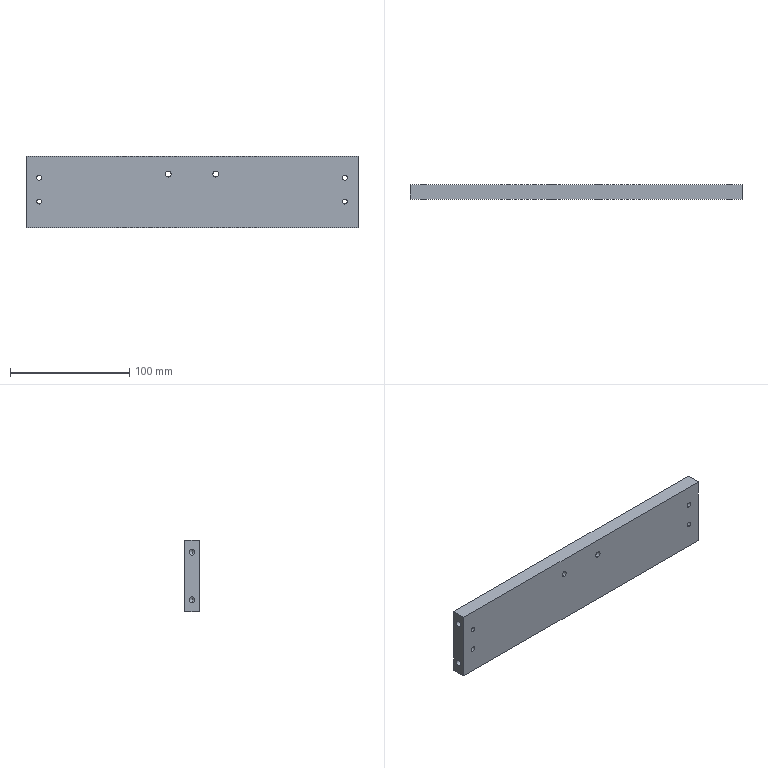Component | SolidWorks | OPW-05-005-1 | 1 solid | 34 faces | box 278 x 12 x 60 mm | volume 197649 mm3 | cylinder 20 | cone 8 | plane 6 | commonest cylinder face diameters 5 x12 4.2 x8
build123d program:
from build123d import *

# Parameters (mm, degrees)
SKETCH1_W                  = 278
SKETCH1_H                  = 60
BOSS_EXTRUDE1_DEPTH        = 6
M6_TAPPED_HOLE1_AT_2_COUNT = 2
M6_TAPPED_HOLE1_AT_2_PITCH = 40
M5_TAPPED_HOLE1_D          = 4.2
M5_TAPPED_HOLE1_DEPTH      = 14
M5_TAPPED_HOLE1_TIP        = 1.262
M6_TAPPED_HOLE2_D          = 5
M6_TAPPED_HOLE2_DEPTH      = 17
M6_TAPPED_HOLE2_TIP        = 1.502


with BuildPart() as part:
    # Sketch1 → Boss-Extrude1 (new, symmetric)
    with BuildSketch(Plane(origin=(0, 0, 0), x_dir=(1, 0, 0), z_dir=(0, 1, 0))):
        Rectangle(SKETCH1_W, SKETCH1_H)
    extrude(amount=BOSS_EXTRUDE1_DEPTH, both=True)

    # Sketch4 → M6 Tapped Hole1 (revolve, cut)
    with BuildSketch(Plane(origin=(-139, 0, -20), x_dir=(0, 0, 1), z_dir=(0, 1, 0))):
        Polygon((0, 0), (0, 18.502), (2.5, 17), (2.5, 0), align=None)
    m6_tapped_hole1 = revolve(axis=Axis((-145.35, 0, -20), (1, 0, 0)), mode=Mode.SUBTRACT)

    # M6 Tapped Hole1 at 2: M6 Tapped Hole1 ×2
    with Locations(*[(0, 0, i * M6_TAPPED_HOLE1_AT_2_PITCH) for i in range(1, M6_TAPPED_HOLE1_AT_2_COUNT)]):
        add(m6_tapped_hole1, mode=Mode.SUBTRACT)

    # Mirror1: M6 Tapped Hole1 across plane
    add(m6_tapped_hole1.mirror(Plane(origin=(0, 0, 0), x_dir=(0, 0, 1), z_dir=(1, 0, 0))), mode=Mode.SUBTRACT)

    # Mirror1 copy 1 sketch → Mirror1 copy 1 (revolve, cut)
    with BuildSketch(Plane(origin=(139, 0, 20), x_dir=(0, 0, 1), z_dir=(0, 1, 0))):
        Polygon((0, 0), (0, -18.502), (2.5, -17), (2.5, 0), align=None)
    revolve(axis=Axis((145.35, 0, 20), (1, 0, 0)), mode=Mode.SUBTRACT)

    # M5 Tapped Hole1
    with Locations(Plane(origin=(0, 6, 0), x_dir=(-1, 0, 0), z_dir=(0, 1, 0))):
        with Locations((128, 12), (128, -8), (-128, -8), (-128, 12)):
            Hole(M5_TAPPED_HOLE1_D / 2, depth=M5_TAPPED_HOLE1_DEPTH)
            with Locations((0, 0, -(M5_TAPPED_HOLE1_DEPTH + M5_TAPPED_HOLE1_TIP / 2))):  # 118° drill point
                Cone(0, M5_TAPPED_HOLE1_D / 2, M5_TAPPED_HOLE1_TIP, mode=Mode.SUBTRACT)

    # M6 Tapped Hole2
    with Locations(Plane(origin=(0, 6, 0), x_dir=(-1, 0, 0), z_dir=(0, 1, 0))):
        with Locations((20, 15), (-20, 15)):
            Hole(M6_TAPPED_HOLE2_D / 2, depth=M6_TAPPED_HOLE2_DEPTH)
            with Locations((0, 0, -(M6_TAPPED_HOLE2_DEPTH + M6_TAPPED_HOLE2_TIP / 2))):  # 118° drill point
                Cone(0, M6_TAPPED_HOLE2_D / 2, M6_TAPPED_HOLE2_TIP, mode=Mode.SUBTRACT)


solid = part.part

# Placed as in the assembly
solid = solid.moved(Location((-104.904, 149.999, 0), (0, 0, 0)))
STEP:
#1=COLOUR_RGB('',0.7922,0.8196,0.9333);
#2=FILL_AREA_STYLE_COLOUR('',#1);
#3=FILL_AREA_STYLE('',(#2));
#4=SURFACE_STYLE_FILL_AREA(#3);
#5=SURFACE_SIDE_STYLE('',(#4));
#6=SURFACE_STYLE_USAGE(.BOTH.,#5);
#7=PRESENTATION_STYLE_ASSIGNMENT((#6));
#8=CARTESIAN_POINT('',(-4.917,5.669,0.4921));
#9=VERTEX_POINT('',#8);
#10=CARTESIAN_POINT('',(-4.917,5.669,0.689));
#11=VERTEX_POINT('',#10);
#12=CARTESIAN_POINT('',(-4.917,5.669,0.5906));
#13=DIRECTION('',(0.,1.,0.));
#14=DIRECTION('',(0.,0.,1.));
#15=AXIS2_PLACEMENT_3D('',#12,#13,#14);
#16=CIRCLE('',#15,0.09843);
#17=EDGE_CURVE('',#9,#11,#16,.T.);
#18=ORIENTED_EDGE('',*,*,#17,.F.);
#19=CARTESIAN_POINT('',(-4.917,6.142,0.4921));
#20=VERTEX_POINT('',#19);
#21=CARTESIAN_POINT('',(-4.917,6.142,0.4921));
#22=DIRECTION('',(0.,1.,0.));
#23=VECTOR('',#22,39.37);
#24=LINE('',#21,#23);
#25=EDGE_CURVE('',#9,#20,#24,.T.);
#26=ORIENTED_EDGE('',*,*,#25,.T.);
#27=CARTESIAN_POINT('',(-4.917,6.142,0.689));
#28=VERTEX_POINT('',#27);
#29=CARTESIAN_POINT('',(-4.917,6.142,0.5906));
#30=DIRECTION('',(0.,1.,0.));
#31=DIRECTION('',(0.,0.,1.));
#32=AXIS2_PLACEMENT_3D('',#29,#30,#31);
#33=CIRCLE('',#32,0.09843);
#34=EDGE_CURVE('',#20,#28,#33,.T.);
#35=ORIENTED_EDGE('',*,*,#34,.T.);
#36=CARTESIAN_POINT('',(-4.917,6.142,0.689));
#37=DIRECTION('',(0.,1.,0.));
#38=VECTOR('',#37,39.37);
#39=LINE('',#36,#38);
#40=EDGE_CURVE('',#11,#28,#39,.T.);
#41=ORIENTED_EDGE('',*,*,#40,.F.);
#42=EDGE_LOOP('',(#18,#26,#35,#41));
#43=FACE_OUTER_BOUND('',#42,.T.);
#44=CARTESIAN_POINT('',(-4.917,6.142,0.5906));
#45=DIRECTION('',(0.,1.,0.));
#46=DIRECTION('',(0.,0.,1.));
#47=AXIS2_PLACEMENT_3D('',#44,#45,#46);
#48=CYLINDRICAL_SURFACE('',#47,0.09843);
#49=ADVANCED_FACE('',(#43),#48,.F.);
#50=CARTESIAN_POINT('',(-3.343,5.669,0.4921));
#51=VERTEX_POINT('',#50);
#52=CARTESIAN_POINT('',(-3.343,5.669,0.689));
#53=VERTEX_POINT('',#52);
#54=CARTESIAN_POINT('',(-3.343,5.669,0.5906));
#55=DIRECTION('',(0.,1.,0.));
#56=DIRECTION('',(0.,0.,1.));
#57=AXIS2_PLACEMENT_3D('',#54,#55,#56);
#58=CIRCLE('',#57,0.09843);
#59=EDGE_CURVE('',#51,#53,#58,.T.);
#60=ORIENTED_EDGE('',*,*,#59,.F.);
#61=CARTESIAN_POINT('',(-3.343,6.142,0.4921));
#62=VERTEX_POINT('',#61);
#63=CARTESIAN_POINT('',(-3.343,6.142,0.4921));
#64=DIRECTION('',(0.,1.,0.));
#65=VECTOR('',#64,39.37);
#66=LINE('',#63,#65);
#67=EDGE_CURVE('',#51,#62,#66,.T.);
#68=ORIENTED_EDGE('',*,*,#67,.T.);
#69=CARTESIAN_POINT('',(-3.343,6.142,0.689));
#70=VERTEX_POINT('',#69);
#71=CARTESIAN_POINT('',(-3.343,6.142,0.5906));
#72=DIRECTION('',(0.,1.,0.));
#73=DIRECTION('',(0.,0.,1.));
#74=AXIS2_PLACEMENT_3D('',#71,#72,#73);
#75=CIRCLE('',#74,0.09843);
#76=EDGE_CURVE('',#62,#70,#75,.T.);
#77=ORIENTED_EDGE('',*,*,#76,.T.);
#78=CARTESIAN_POINT('',(-3.343,6.142,0.689));
#79=DIRECTION('',(0.,1.,0.));
#80=VECTOR('',#79,39.37);
#81=LINE('',#78,#80);
#82=EDGE_CURVE('',#53,#70,#81,.T.);
#83=ORIENTED_EDGE('',*,*,#82,.F.);
#84=EDGE_LOOP('',(#60,#68,#77,#83));
#85=FACE_OUTER_BOUND('',#84,.T.);
#86=CARTESIAN_POINT('',(-3.343,6.142,0.5906));
#87=DIRECTION('',(0.,1.,0.));
#88=DIRECTION('',(0.,0.,1.));
#89=AXIS2_PLACEMENT_3D('',#86,#87,#88);
#90=CYLINDRICAL_SURFACE('',#89,0.09843);
#91=ADVANCED_FACE('',(#85),#90,.F.);
#92=CARTESIAN_POINT('',(-9.169,5.669,0.3898));
#93=VERTEX_POINT('',#92);
#94=CARTESIAN_POINT('',(-9.169,5.669,0.5551));
#95=VERTEX_POINT('',#94);
#96=CARTESIAN_POINT('',(-9.169,5.669,0.4724));
#97=DIRECTION('',(0.,1.,0.));
#98=DIRECTION('',(0.,0.,1.));
#99=AXIS2_PLACEMENT_3D('',#96,#97,#98);
#100=CIRCLE('',#99,0.08268);
#101=EDGE_CURVE('',#93,#95,#100,.T.);
#102=ORIENTED_EDGE('',*,*,#101,.F.);
#103=CARTESIAN_POINT('',(-9.169,6.142,0.3898));
#104=VERTEX_POINT('',#103);
#105=CARTESIAN_POINT('',(-9.169,6.142,0.3898));
#106=DIRECTION('',(0.,1.,0.));
#107=VECTOR('',#106,39.37);
#108=LINE('',#105,#107);
#109=EDGE_CURVE('',#93,#104,#108,.T.);
#110=ORIENTED_EDGE('',*,*,#109,.T.);
#111=CARTESIAN_POINT('',(-9.169,6.142,0.5551));
#112=VERTEX_POINT('',#111);
#113=CARTESIAN_POINT('',(-9.169,6.142,0.4724));
#114=DIRECTION('',(0.,1.,0.));
#115=DIRECTION('',(0.,0.,1.));
#116=AXIS2_PLACEMENT_3D('',#113,#114,#115);
#117=CIRCLE('',#116,0.08268);
#118=EDGE_CURVE('',#104,#112,#117,.T.);
#119=ORIENTED_EDGE('',*,*,#118,.T.);
#120=CARTESIAN_POINT('',(-9.169,6.142,0.5551));
#121=DIRECTION('',(0.,1.,0.));
#122=VECTOR('',#121,39.37);
#123=LINE('',#120,#122);
#124=EDGE_CURVE('',#95,#112,#123,.T.);
#125=ORIENTED_EDGE('',*,*,#124,.F.);
#126=EDGE_LOOP('',(#102,#110,#119,#125));
#127=FACE_OUTER_BOUND('',#126,.T.);
#128=CARTESIAN_POINT('',(-9.169,6.142,0.4724));
#129=DIRECTION('',(0.,1.,0.));
#130=DIRECTION('',(0.,0.,1.));
#131=AXIS2_PLACEMENT_3D('',#128,#129,#130);
#132=CYLINDRICAL_SURFACE('',#131,0.08268);
#133=ADVANCED_FACE('',(#127),#132,.F.);
#134=CARTESIAN_POINT('',(-9.169,5.669,-0.3976));
#135=VERTEX_POINT('',#134);
#136=CARTESIAN_POINT('',(-9.169,5.669,-0.2323));
#137=VERTEX_POINT('',#136);
#138=CARTESIAN_POINT('',(-9.169,5.669,-0.315));
#139=DIRECTION('',(0.,1.,0.));
#140=DIRECTION('',(0.,0.,1.));
#141=AXIS2_PLACEMENT_3D('',#138,#139,#140);
#142=CIRCLE('',#141,0.08268);
#143=EDGE_CURVE('',#135,#137,#142,.T.);
#144=ORIENTED_EDGE('',*,*,#143,.F.);
#145=CARTESIAN_POINT('',(-9.169,6.142,-0.3976));
#146=VERTEX_POINT('',#145);
#147=CARTESIAN_POINT('',(-9.169,6.142,-0.3976));
#148=DIRECTION('',(0.,1.,0.));
#149=VECTOR('',#148,39.37);
#150=LINE('',#147,#149);
#151=EDGE_CURVE('',#135,#146,#150,.T.);
#152=ORIENTED_EDGE('',*,*,#151,.T.);
#153=CARTESIAN_POINT('',(-9.169,6.142,-0.2323));
#154=VERTEX_POINT('',#153);
#155=CARTESIAN_POINT('',(-9.169,6.142,-0.315));
#156=DIRECTION('',(0.,1.,0.));
#157=DIRECTION('',(0.,0.,1.));
#158=AXIS2_PLACEMENT_3D('',#155,#156,#157);
#159=CIRCLE('',#158,0.08268);
#160=EDGE_CURVE('',#146,#154,#159,.T.);
#161=ORIENTED_EDGE('',*,*,#160,.T.);
#162=CARTESIAN_POINT('',(-9.169,6.142,-0.2323));
#163=DIRECTION('',(0.,1.,0.));
#164=VECTOR('',#163,39.37);
#165=LINE('',#162,#164);
#166=EDGE_CURVE('',#137,#154,#165,.T.);
#167=ORIENTED_EDGE('',*,*,#166,.F.);
#168=EDGE_LOOP('',(#144,#152,#161,#167));
#169=FACE_OUTER_BOUND('',#168,.T.);
#170=CARTESIAN_POINT('',(-9.169,6.142,-0.315));
#171=DIRECTION('',(0.,1.,0.));
#172=DIRECTION('',(0.,0.,1.));
#173=AXIS2_PLACEMENT_3D('',#170,#171,#172);
#174=CYLINDRICAL_SURFACE('',#173,0.08268);
#175=ADVANCED_FACE('',(#169),#174,.F.);
#176=CARTESIAN_POINT('',(0.9093,5.669,-0.3976));
#177=VERTEX_POINT('',#176);
#178=CARTESIAN_POINT('',(0.9093,5.669,-0.2323));
#179=VERTEX_POINT('',#178);
#180=CARTESIAN_POINT('',(0.9093,5.669,-0.315));
#181=DIRECTION('',(0.,1.,0.));
#182=DIRECTION('',(0.,0.,1.));
#183=AXIS2_PLACEMENT_3D('',#180,#181,#182);
#184=CIRCLE('',#183,0.08268);
#185=EDGE_CURVE('',#177,#179,#184,.T.);
#186=ORIENTED_EDGE('',*,*,#185,.F.);
#187=CARTESIAN_POINT('',(0.9093,6.142,-0.3976));
#188=VERTEX_POINT('',#187);
#189=CARTESIAN_POINT('',(0.9093,6.142,-0.3976));
#190=DIRECTION('',(0.,1.,0.));
#191=VECTOR('',#190,39.37);
#192=LINE('',#189,#191);
#193=EDGE_CURVE('',#177,#188,#192,.T.);
#194=ORIENTED_EDGE('',*,*,#193,.T.);
#195=CARTESIAN_POINT('',(0.9093,6.142,-0.2323));
#196=VERTEX_POINT('',#195);
#197=CARTESIAN_POINT('',(0.9093,6.142,-0.315));
#198=DIRECTION('',(0.,1.,0.));
#199=DIRECTION('',(0.,0.,1.));
#200=AXIS2_PLACEMENT_3D('',#197,#198,#199);
#201=CIRCLE('',#200,0.08268);
#202=EDGE_CURVE('',#188,#196,#201,.T.);
#203=ORIENTED_EDGE('',*,*,#202,.T.);
#204=CARTESIAN_POINT('',(0.9093,6.142,-0.2323));
#205=DIRECTION('',(0.,1.,0.));
#206=VECTOR('',#205,39.37);
#207=LINE('',#204,#206);
#208=EDGE_CURVE('',#179,#196,#207,.T.);
#209=ORIENTED_EDGE('',*,*,#208,.F.);
#210=EDGE_LOOP('',(#186,#194,#203,#209));
#211=FACE_OUTER_BOUND('',#210,.T.);
#212=CARTESIAN_POINT('',(0.9093,6.142,-0.315));
#213=DIRECTION('',(0.,1.,0.));
#214=DIRECTION('',(0.,0.,1.));
#215=AXIS2_PLACEMENT_3D('',#212,#213,#214);
#216=CYLINDRICAL_SURFACE('',#215,0.08268);
#217=ADVANCED_FACE('',(#211),#216,.F.);
#218=CARTESIAN_POINT('',(0.9093,5.669,0.3898));
#219=VERTEX_POINT('',#218);
#220=CARTESIAN_POINT('',(0.9093,5.669,0.5551));
#221=VERTEX_POINT('',#220);
#222=CARTESIAN_POINT('',(0.9093,5.669,0.4724));
#223=DIRECTION('',(0.,1.,0.));
#224=DIRECTION('',(0.,0.,1.));
#225=AXIS2_PLACEMENT_3D('',#222,#223,#224);
#226=CIRCLE('',#225,0.08268);
#227=EDGE_CURVE('',#219,#221,#226,.T.);
#228=ORIENTED_EDGE('',*,*,#227,.F.);
#229=CARTESIAN_POINT('',(0.9093,6.142,0.3898));
#230=VERTEX_POINT('',#229);
#231=CARTESIAN_POINT('',(0.9093,6.142,0.3898));
#232=DIRECTION('',(0.,1.,0.));
#233=VECTOR('',#232,39.37);
#234=LINE('',#231,#233);
#235=EDGE_CURVE('',#219,#230,#234,.T.);
#236=ORIENTED_EDGE('',*,*,#235,.T.);
#237=CARTESIAN_POINT('',(0.9093,6.142,0.5551));
#238=VERTEX_POINT('',#237);
#239=CARTESIAN_POINT('',(0.9093,6.142,0.4724));
#240=DIRECTION('',(0.,1.,0.));
#241=DIRECTION('',(0.,0.,1.));
#242=AXIS2_PLACEMENT_3D('',#239,#240,#241);
#243=CIRCLE('',#242,0.08268);
#244=EDGE_CURVE('',#230,#238,#243,.T.);
#245=ORIENTED_EDGE('',*,*,#244,.T.);
#246=CARTESIAN_POINT('',(0.9093,6.142,0.5551));
#247=DIRECTION('',(0.,1.,0.));
#248=VECTOR('',#247,39.37);
#249=LINE('',#246,#248);
#250=EDGE_CURVE('',#221,#238,#249,.T.);
#251=ORIENTED_EDGE('',*,*,#250,.F.);
#252=EDGE_LOOP('',(#228,#236,#245,#251));
#253=FACE_OUTER_BOUND('',#252,.T.);
#254=CARTESIAN_POINT('',(0.9093,6.142,0.4724));
#255=DIRECTION('',(0.,1.,0.));
#256=DIRECTION('',(0.,0.,1.));
#257=AXIS2_PLACEMENT_3D('',#254,#255,#256);
#258=CYLINDRICAL_SURFACE('',#257,0.08268);
#259=ADVANCED_FACE('',(#253),#258,.F.);
#260=CARTESIAN_POINT('',(0.6731,5.905,-0.689));
#261=VERTEX_POINT('',#260);
#262=CARTESIAN_POINT('',(0.6731,5.905,-0.8858));
#263=VERTEX_POINT('',#262);
#264=CARTESIAN_POINT('',(0.6731,5.905,-0.7874));
#265=DIRECTION('',(1.,0.,0.));
#266=DIRECTION('',(0.,0.,-1.));
#267=AXIS2_PLACEMENT_3D('',#264,#265,#266);
#268=CIRCLE('',#267,0.09843);
#269=EDGE_CURVE('',#261,#263,#268,.T.);
#270=ORIENTED_EDGE('',*,*,#269,.F.);
#271=CARTESIAN_POINT('',(1.342,5.905,-0.689));
#272=VERTEX_POINT('',#271);
#273=CARTESIAN_POINT('',(1.342,5.905,-0.689));
#274=DIRECTION('',(1.,0.,0.));
#275=VECTOR('',#274,39.37);
#276=LINE('',#273,#275);
#277=EDGE_CURVE('',#261,#272,#276,.T.);
#278=ORIENTED_EDGE('',*,*,#277,.T.);
#279=CARTESIAN_POINT('',(1.342,5.905,-0.8858));
#280=VERTEX_POINT('',#279);
#281=CARTESIAN_POINT('',(1.342,5.905,-0.7874));
#282=DIRECTION('',(1.,0.,0.));
#283=DIRECTION('',(0.,0.,-1.));
#284=AXIS2_PLACEMENT_3D('',#281,#282,#283);
#285=CIRCLE('',#284,0.09843);
#286=EDGE_CURVE('',#272,#280,#285,.T.);
#287=ORIENTED_EDGE('',*,*,#286,.T.);
#288=CARTESIAN_POINT('',(1.342,5.905,-0.8858));
#289=DIRECTION('',(1.,0.,0.));
#290=VECTOR('',#289,39.37);
#291=LINE('',#288,#290);
#292=EDGE_CURVE('',#263,#280,#291,.T.);
#293=ORIENTED_EDGE('',*,*,#292,.F.);
#294=EDGE_LOOP('',(#270,#278,#287,#293));
#295=FACE_OUTER_BOUND('',#294,.T.);
#296=CARTESIAN_POINT('',(1.342,5.905,-0.7874));
#297=DIRECTION('',(1.,0.,0.));
#298=DIRECTION('',(0.,0.,-1.));
#299=AXIS2_PLACEMENT_3D('',#296,#297,#298);
#300=CYLINDRICAL_SURFACE('',#299,0.09843);
#301=ADVANCED_FACE('',(#295),#300,.F.);
#302=CARTESIAN_POINT('',(0.6139,5.905,-0.7874));
#303=VERTEX_POINT('',#302);
#304=CARTESIAN_POINT('',(0.6731,5.905,-0.8858));
#305=DIRECTION('',(0.515,0.,-0.8572));
#306=VECTOR('',#305,39.37);
#307=LINE('',#304,#306);
#308=EDGE_CURVE('',#303,#263,#307,.T.);
#309=ORIENTED_EDGE('',*,*,#308,.F.);
#310=CARTESIAN_POINT('',(0.6731,5.905,-0.689));
#311=DIRECTION('',(0.515,0.,0.8572));
#312=VECTOR('',#311,39.37);
#313=LINE('',#310,#312);
#314=EDGE_CURVE('',#303,#261,#313,.T.);
#315=ORIENTED_EDGE('',*,*,#314,.T.);
#316=ORIENTED_EDGE('',*,*,#269,.T.);
#317=EDGE_LOOP('',(#309,#315,#316));
#318=FACE_OUTER_BOUND('',#317,.T.);
#319=CARTESIAN_POINT('',(0.6731,5.905,-0.7874));
#320=DIRECTION('',(1.,0.,0.));
#321=DIRECTION('',(0.,0.,-1.));
#322=AXIS2_PLACEMENT_3D('',#319,#320,#321);
#323=CONICAL_SURFACE('',#322,0.09843,1.03);
#324=ADVANCED_FACE('',(#318),#323,.F.);
#325=CARTESIAN_POINT('',(0.6731,5.905,0.8858));
#326=VERTEX_POINT('',#325);
#327=CARTESIAN_POINT('',(0.6731,5.905,0.689));
#328=VERTEX_POINT('',#327);
#329=CARTESIAN_POINT('',(0.6731,5.905,0.7874));
#330=DIRECTION('',(1.,0.,0.));
#331=DIRECTION('',(0.,0.,-1.));
#332=AXIS2_PLACEMENT_3D('',#329,#330,#331);
#333=CIRCLE('',#332,0.09843);
#334=EDGE_CURVE('',#326,#328,#333,.T.);
#335=ORIENTED_EDGE('',*,*,#334,.F.);
#336=CARTESIAN_POINT('',(1.342,5.905,0.8858));
#337=VERTEX_POINT('',#336);
#338=CARTESIAN_POINT('',(1.342,5.905,0.8858));
#339=DIRECTION('',(1.,0.,0.));
#340=VECTOR('',#339,39.37);
#341=LINE('',#338,#340);
#342=EDGE_CURVE('',#326,#337,#341,.T.);
#343=ORIENTED_EDGE('',*,*,#342,.T.);
#344=CARTESIAN_POINT('',(1.342,5.905,0.689));
#345=VERTEX_POINT('',#344);
#346=CARTESIAN_POINT('',(1.342,5.905,0.7874));
#347=DIRECTION('',(1.,0.,0.));
#348=DIRECTION('',(0.,0.,-1.));
#349=AXIS2_PLACEMENT_3D('',#346,#347,#348);
#350=CIRCLE('',#349,0.09843);
#351=EDGE_CURVE('',#337,#345,#350,.T.);
#352=ORIENTED_EDGE('',*,*,#351,.T.);
#353=CARTESIAN_POINT('',(1.342,5.905,0.689));
#354=DIRECTION('',(1.,0.,0.));
#355=VECTOR('',#354,39.37);
#356=LINE('',#353,#355);
#357=EDGE_CURVE('',#328,#345,#356,.T.);
#358=ORIENTED_EDGE('',*,*,#357,.F.);
#359=EDGE_LOOP('',(#335,#343,#352,#358));
#360=FACE_OUTER_BOUND('',#359,.T.);
#361=CARTESIAN_POINT('',(1.342,5.905,0.7874));
#362=DIRECTION('',(1.,0.,0.));
#363=DIRECTION('',(0.,0.,-1.));
#364=AXIS2_PLACEMENT_3D('',#361,#362,#363);
#365=CYLINDRICAL_SURFACE('',#364,0.09843);
#366=ADVANCED_FACE('',(#360),#365,.F.);
#367=CARTESIAN_POINT('',(0.6139,5.905,0.7874));
#368=VERTEX_POINT('',#367);
#369=CARTESIAN_POINT('',(0.6731,5.905,0.689));
#370=DIRECTION('',(0.515,0.,-0.8572));
#371=VECTOR('',#370,39.37);
#372=LINE('',#369,#371);
#373=EDGE_CURVE('',#368,#328,#372,.T.);
#374=ORIENTED_EDGE('',*,*,#373,.F.);
#375=CARTESIAN_POINT('',(0.6731,5.905,0.8858));
#376=DIRECTION('',(0.515,0.,0.8572));
#377=VECTOR('',#376,39.37);
#378=LINE('',#375,#377);
#379=EDGE_CURVE('',#368,#326,#378,.T.);
#380=ORIENTED_EDGE('',*,*,#379,.T.);
#381=ORIENTED_EDGE('',*,*,#334,.T.);
#382=EDGE_LOOP('',(#374,#380,#381));
#383=FACE_OUTER_BOUND('',#382,.T.);
#384=CARTESIAN_POINT('',(0.6731,5.905,0.7874));
#385=DIRECTION('',(1.,0.,0.));
#386=DIRECTION('',(0.,0.,-1.));
#387=AXIS2_PLACEMENT_3D('',#384,#385,#386);
#388=CONICAL_SURFACE('',#387,0.09843,1.03);
#389=ADVANCED_FACE('',(#383),#388,.F.);
#390=CARTESIAN_POINT('',(-8.933,5.905,-0.8858));
#391=VERTEX_POINT('',#390);
#392=CARTESIAN_POINT('',(-8.933,5.905,-0.689));
#393=VERTEX_POINT('',#392);
#394=CARTESIAN_POINT('',(-8.933,5.905,-0.7874));
#395=DIRECTION('',(-1.,0.,0.));
#396=DIRECTION('',(0.,0.,1.));
#397=AXIS2_PLACEMENT_3D('',#394,#395,#396);
#398=CIRCLE('',#397,0.09843);
#399=EDGE_CURVE('',#391,#393,#398,.T.);
#400=ORIENTED_EDGE('',*,*,#399,.F.);
#401=CARTESIAN_POINT('',(-9.603,5.905,-0.8858));
#402=VERTEX_POINT('',#401);
#403=CARTESIAN_POINT('',(-9.603,5.905,-0.8858));
#404=DIRECTION('',(-1.,0.,0.));
#405=VECTOR('',#404,39.37);
#406=LINE('',#403,#405);
#407=EDGE_CURVE('',#391,#402,#406,.T.);
#408=ORIENTED_EDGE('',*,*,#407,.T.);
#409=CARTESIAN_POINT('',(-9.603,5.905,-0.689));
#410=VERTEX_POINT('',#409);
#411=CARTESIAN_POINT('',(-9.603,5.905,-0.7874));
#412=DIRECTION('',(-1.,0.,0.));
#413=DIRECTION('',(0.,0.,1.));
#414=AXIS2_PLACEMENT_3D('',#411,#412,#413);
#415=CIRCLE('',#414,0.09843);
#416=EDGE_CURVE('',#402,#410,#415,.T.);
#417=ORIENTED_EDGE('',*,*,#416,.T.);
#418=CARTESIAN_POINT('',(-9.603,5.905,-0.689));
#419=DIRECTION('',(-1.,0.,0.));
#420=VECTOR('',#419,39.37);
#421=LINE('',#418,#420);
#422=EDGE_CURVE('',#393,#410,#421,.T.);
#423=ORIENTED_EDGE('',*,*,#422,.F.);
#424=EDGE_LOOP('',(#400,#408,#417,#423));
#425=FACE_OUTER_BOUND('',#424,.T.);
#426=CARTESIAN_POINT('',(-9.603,5.905,-0.7874));
#427=DIRECTION('',(-1.,0.,0.));
#428=DIRECTION('',(0.,0.,1.));
#429=AXIS2_PLACEMENT_3D('',#426,#427,#428);
#430=CYLINDRICAL_SURFACE('',#429,0.09843);
#431=ADVANCED_FACE('',(#425),#430,.F.);
#432=CARTESIAN_POINT('',(-8.874,5.905,-0.7874));
#433=VERTEX_POINT('',#432);
#434=CARTESIAN_POINT('',(-8.933,5.905,-0.689));
#435=DIRECTION('',(-0.515,0.,0.8572));
#436=VECTOR('',#435,39.37);
#437=LINE('',#434,#436);
#438=EDGE_CURVE('',#433,#393,#437,.T.);
#439=ORIENTED_EDGE('',*,*,#438,.F.);
#440=CARTESIAN_POINT('',(-8.933,5.905,-0.8858));
#441=DIRECTION('',(-0.515,0.,-0.8572));
#442=VECTOR('',#441,39.37);
#443=LINE('',#440,#442);
#444=EDGE_CURVE('',#433,#391,#443,.T.);
#445=ORIENTED_EDGE('',*,*,#444,.T.);
#446=ORIENTED_EDGE('',*,*,#399,.T.);
#447=EDGE_LOOP('',(#439,#445,#446));
#448=FACE_OUTER_BOUND('',#447,.T.);
#449=CARTESIAN_POINT('',(-8.933,5.905,-0.7874));
#450=DIRECTION('',(-1.,0.,0.));
#451=DIRECTION('',(0.,0.,1.));
#452=AXIS2_PLACEMENT_3D('',#449,#450,#451);
#453=CONICAL_SURFACE('',#452,0.09843,1.03);
#454=ADVANCED_FACE('',(#448),#453,.F.);
#455=CARTESIAN_POINT('',(-8.933,5.905,0.689));
#456=VERTEX_POINT('',#455);
#457=CARTESIAN_POINT('',(-8.933,5.905,0.8858));
#458=VERTEX_POINT('',#457);
#459=CARTESIAN_POINT('',(-8.933,5.905,0.7874));
#460=DIRECTION('',(-1.,0.,0.));
#461=DIRECTION('',(0.,0.,1.));
#462=AXIS2_PLACEMENT_3D('',#459,#460,#461);
#463=CIRCLE('',#462,0.09843);
#464=EDGE_CURVE('',#456,#458,#463,.T.);
#465=ORIENTED_EDGE('',*,*,#464,.F.);
#466=CARTESIAN_POINT('',(-9.603,5.905,0.689));
#467=VERTEX_POINT('',#466);
#468=CARTESIAN_POINT('',(-9.603,5.905,0.689));
#469=DIRECTION('',(-1.,0.,0.));
#470=VECTOR('',#469,39.37);
#471=LINE('',#468,#470);
#472=EDGE_CURVE('',#456,#467,#471,.T.);
#473=ORIENTED_EDGE('',*,*,#472,.T.);
#474=CARTESIAN_POINT('',(-9.603,5.905,0.8858));
#475=VERTEX_POINT('',#474);
#476=CARTESIAN_POINT('',(-9.603,5.905,0.7874));
#477=DIRECTION('',(-1.,0.,0.));
#478=DIRECTION('',(0.,0.,1.));
#479=AXIS2_PLACEMENT_3D('',#476,#477,#478);
#480=CIRCLE('',#479,0.09843);
#481=EDGE_CURVE('',#467,#475,#480,.T.);
#482=ORIENTED_EDGE('',*,*,#481,.T.);
#483=CARTESIAN_POINT('',(-9.603,5.905,0.8858));
#484=DIRECTION('',(-1.,0.,0.));
#485=VECTOR('',#484,39.37);
#486=LINE('',#483,#485);
#487=EDGE_CURVE('',#458,#475,#486,.T.);
#488=ORIENTED_EDGE('',*,*,#487,.F.);
#489=EDGE_LOOP('',(#465,#473,#482,#488));
#490=FACE_OUTER_BOUND('',#489,.T.);
#491=CARTESIAN_POINT('',(-9.603,5.905,0.7874));
#492=DIRECTION('',(-1.,0.,0.));
#493=DIRECTION('',(0.,0.,1.));
#494=AXIS2_PLACEMENT_3D('',#491,#492,#493);
#495=CYLINDRICAL_SURFACE('',#494,0.09843);
#496=ADVANCED_FACE('',(#490),#495,.F.);
#497=CARTESIAN_POINT('',(-8.874,5.905,0.7874));
#498=VERTEX_POINT('',#497);
#499=CARTESIAN_POINT('',(-8.933,5.905,0.8858));
#500=DIRECTION('',(-0.515,0.,0.8572));
#501=VECTOR('',#500,39.37);
#502=LINE('',#499,#501);
#503=EDGE_CURVE('',#498,#458,#502,.T.);
#504=ORIENTED_EDGE('',*,*,#503,.F.);
#505=CARTESIAN_POINT('',(-8.933,5.905,0.689));
#506=DIRECTION('',(-0.515,0.,-0.8572));
#507=VECTOR('',#506,39.37);
#508=LINE('',#505,#507);
#509=EDGE_CURVE('',#498,#456,#508,.T.);
#510=ORIENTED_EDGE('',*,*,#509,.T.);
#511=ORIENTED_EDGE('',*,*,#464,.T.);
#512=EDGE_LOOP('',(#504,#510,#511));
#513=FACE_OUTER_BOUND('',#512,.T.);
#514=CARTESIAN_POINT('',(-8.933,5.905,0.7874));
#515=DIRECTION('',(-1.,0.,0.));
#516=DIRECTION('',(0.,0.,1.));
#517=AXIS2_PLACEMENT_3D('',#514,#515,#516);
#518=CONICAL_SURFACE('',#517,0.09843,1.03);
#519=ADVANCED_FACE('',(#513),#518,.F.);
#520=CARTESIAN_POINT('',(1.342,5.905,0.7874));
#521=DIRECTION('',(1.,0.,0.));
#522=DIRECTION('',(0.,0.,-1.));
#523=AXIS2_PLACEMENT_3D('',#520,#521,#522);
#524=CIRCLE('',#523,0.09843);
#525=EDGE_CURVE('',#345,#337,#524,.T.);
#526=ORIENTED_EDGE('',*,*,#525,.F.);
#527=ORIENTED_EDGE('',*,*,#351,.F.);
#528=EDGE_LOOP('',(#526,#527));
#529=FACE_BOUND('',#528,.T.);
#530=CARTESIAN_POINT('',(1.342,5.669,1.181));
#531=VERTEX_POINT('',#530);
#532=CARTESIAN_POINT('',(1.342,5.669,-1.181));
#533=VERTEX_POINT('',#532);
#534=CARTESIAN_POINT('',(1.342,5.669,-1.181));
#535=DIRECTION('',(0.,0.,-1.));
#536=VECTOR('',#535,39.37);
#537=LINE('',#534,#536);
#538=EDGE_CURVE('',#531,#533,#537,.T.);
#539=ORIENTED_EDGE('',*,*,#538,.T.);
#540=CARTESIAN_POINT('',(1.342,6.142,-1.181));
#541=VERTEX_POINT('',#540);
#542=CARTESIAN_POINT('',(1.342,6.142,-1.181));
#543=DIRECTION('',(0.,-1.,0.));
#544=VECTOR('',#543,39.37);
#545=LINE('',#542,#544);
#546=EDGE_CURVE('',#541,#533,#545,.T.);
#547=ORIENTED_EDGE('',*,*,#546,.F.);
#548=CARTESIAN_POINT('',(1.342,6.142,1.181));
#549=VERTEX_POINT('',#548);
#550=CARTESIAN_POINT('',(1.342,6.142,-1.181));
#551=DIRECTION('',(0.,0.,-1.));
#552=VECTOR('',#551,39.37);
#553=LINE('',#550,#552);
#554=EDGE_CURVE('',#549,#541,#553,.T.);
#555=ORIENTED_EDGE('',*,*,#554,.F.);
#556=CARTESIAN_POINT('',(1.342,6.142,1.181));
#557=DIRECTION('',(0.,-1.,0.));
#558=VECTOR('',#557,39.37);
#559=LINE('',#556,#558);
#560=EDGE_CURVE('',#549,#531,#559,.T.);
#561=ORIENTED_EDGE('',*,*,#560,.T.);
#562=EDGE_LOOP('',(#539,#547,#555,#561));
#563=FACE_OUTER_BOUND('',#562,.T.);
#564=CARTESIAN_POINT('',(1.342,5.905,-0.7874));
#565=DIRECTION('',(1.,0.,0.));
#566=DIRECTION('',(0.,0.,-1.));
#567=AXIS2_PLACEMENT_3D('',#564,#565,#566);
#568=CIRCLE('',#567,0.09843);
#569=EDGE_CURVE('',#280,#272,#568,.T.);
#570=ORIENTED_EDGE('',*,*,#569,.F.);
#571=ORIENTED_EDGE('',*,*,#286,.F.);
#572=EDGE_LOOP('',(#570,#571));
#573=FACE_BOUND('',#572,.T.);
#574=CARTESIAN_POINT('',(1.342,6.142,-1.181));
#575=DIRECTION('',(-1.,0.,0.));
#576=DIRECTION('',(0.,0.,1.));
#577=AXIS2_PLACEMENT_3D('',#574,#575,#576);
#578=PLANE('',#577);
#579=ADVANCED_FACE('',(#529,#563,#573),#578,.F.);
#580=CARTESIAN_POINT('',(-9.603,5.905,-0.7874));
#581=DIRECTION('',(-1.,0.,0.));
#582=DIRECTION('',(0.,0.,1.));
#583=AXIS2_PLACEMENT_3D('',#580,#581,#582);
#584=CIRCLE('',#583,0.09843);
#585=EDGE_CURVE('',#410,#402,#584,.T.);
#586=ORIENTED_EDGE('',*,*,#585,.F.);
#587=ORIENTED_EDGE('',*,*,#416,.F.);
#588=EDGE_LOOP('',(#586,#587));
#589=FACE_BOUND('',#588,.T.);
#590=CARTESIAN_POINT('',(-9.603,5.905,0.7874));
#591=DIRECTION('',(-1.,0.,0.));
#592=DIRECTION('',(0.,0.,1.));
#593=AXIS2_PLACEMENT_3D('',#590,#591,#592);
#594=CIRCLE('',#593,0.09843);
#595=EDGE_CURVE('',#475,#467,#594,.T.);
#596=ORIENTED_EDGE('',*,*,#595,.F.);
#597=ORIENTED_EDGE('',*,*,#481,.F.);
#598=EDGE_LOOP('',(#596,#597));
#599=FACE_BOUND('',#598,.T.);
#600=CARTESIAN_POINT('',(-9.603,5.669,-1.181));
#601=VERTEX_POINT('',#600);
#602=CARTESIAN_POINT('',(-9.603,5.669,1.181));
#603=VERTEX_POINT('',#602);
#604=CARTESIAN_POINT('',(-9.603,5.669,-1.181));
#605=DIRECTION('',(0.,0.,1.));
#606=VECTOR('',#605,39.37);
#607=LINE('',#604,#606);
#608=EDGE_CURVE('',#601,#603,#607,.T.);
#609=ORIENTED_EDGE('',*,*,#608,.T.);
#610=CARTESIAN_POINT('',(-9.603,6.142,1.181));
#611=VERTEX_POINT('',#610);
#612=CARTESIAN_POINT('',(-9.603,6.142,1.181));
#613=DIRECTION('',(0.,-1.,0.));
#614=VECTOR('',#613,39.37);
#615=LINE('',#612,#614);
#616=EDGE_CURVE('',#611,#603,#615,.T.);
#617=ORIENTED_EDGE('',*,*,#616,.F.);
#618=CARTESIAN_POINT('',(-9.603,6.142,-1.181));
#619=VERTEX_POINT('',#618);
#620=CARTESIAN_POINT('',(-9.603,6.142,-1.181));
#621=DIRECTION('',(0.,0.,1.));
#622=VECTOR('',#621,39.37);
#623=LINE('',#620,#622);
#624=EDGE_CURVE('',#619,#611,#623,.T.);
#625=ORIENTED_EDGE('',*,*,#624,.F.);
#626=CARTESIAN_POINT('',(-9.603,6.142,-1.181));
#627=DIRECTION('',(0.,-1.,0.));
#628=VECTOR('',#627,39.37);
#629=LINE('',#626,#628);
#630=EDGE_CURVE('',#619,#601,#629,.T.);
#631=ORIENTED_EDGE('',*,*,#630,.T.);
#632=EDGE_LOOP('',(#609,#617,#625,#631));
#633=FACE_OUTER_BOUND('',#632,.T.);
#634=CARTESIAN_POINT('',(-9.603,6.142,-1.181));
#635=DIRECTION('',(1.,0.,0.));
#636=DIRECTION('',(0.,0.,-1.));
#637=AXIS2_PLACEMENT_3D('',#634,#635,#636);
#638=PLANE('',#637);
#639=ADVANCED_FACE('',(#589,#599,#633),#638,.F.);
#640=CARTESIAN_POINT('',(-9.603,5.669,1.181));
#641=DIRECTION('',(1.,0.,-0.));
#642=VECTOR('',#641,39.37);
#643=LINE('',#640,#642);
#644=EDGE_CURVE('',#603,#531,#643,.T.);
#645=ORIENTED_EDGE('',*,*,#644,.T.);
#646=ORIENTED_EDGE('',*,*,#560,.F.);
#647=CARTESIAN_POINT('',(-9.603,6.142,1.181));
#648=DIRECTION('',(1.,0.,-0.));
#649=VECTOR('',#648,39.37);
#650=LINE('',#647,#649);
#651=EDGE_CURVE('',#611,#549,#650,.T.);
#652=ORIENTED_EDGE('',*,*,#651,.F.);
#653=ORIENTED_EDGE('',*,*,#616,.T.);
#654=EDGE_LOOP('',(#645,#646,#652,#653));
#655=FACE_OUTER_BOUND('',#654,.T.);
#656=CARTESIAN_POINT('',(-9.603,6.142,1.181));
#657=DIRECTION('',(-0.,0.,-1.));
#658=DIRECTION('',(-1.,0.,0.));
#659=AXIS2_PLACEMENT_3D('',#656,#657,#658);
#660=PLANE('',#659);
#661=ADVANCED_FACE('',(#655),#660,.F.);
#662=CARTESIAN_POINT('',(-9.603,5.669,-1.181));
#663=DIRECTION('',(-1.,0.,-0.));
#664=VECTOR('',#663,39.37);
#665=LINE('',#662,#664);
#666=EDGE_CURVE('',#533,#601,#665,.T.);
#667=ORIENTED_EDGE('',*,*,#666,.T.);
#668=ORIENTED_EDGE('',*,*,#630,.F.);
#669=CARTESIAN_POINT('',(-9.603,6.142,-1.181));
#670=DIRECTION('',(-1.,0.,-0.));
#671=VECTOR('',#670,39.37);
#672=LINE('',#669,#671);
#673=EDGE_CURVE('',#541,#619,#672,.T.);
#674=ORIENTED_EDGE('',*,*,#673,.F.);
#675=ORIENTED_EDGE('',*,*,#546,.T.);
#676=EDGE_LOOP('',(#667,#668,#674,#675));
#677=FACE_OUTER_BOUND('',#676,.T.);
#678=CARTESIAN_POINT('',(-9.603,6.142,-1.181));
#679=DIRECTION('',(-0.,0.,1.));
#680=DIRECTION('',(1.,0.,0.));
#681=AXIS2_PLACEMENT_3D('',#678,#679,#680);
#682=PLANE('',#681);
#683=ADVANCED_FACE('',(#677),#682,.F.);
#684=CARTESIAN_POINT('',(-4.917,6.142,0.5906));
#685=DIRECTION('',(0.,1.,0.));
#686=DIRECTION('',(0.,0.,1.));
#687=AXIS2_PLACEMENT_3D('',#684,#685,#686);
#688=CIRCLE('',#687,0.09843);
#689=EDGE_CURVE('',#28,#20,#688,.T.);
#690=ORIENTED_EDGE('',*,*,#689,.F.);
#691=ORIENTED_EDGE('',*,*,#34,.F.);
#692=EDGE_LOOP('',(#690,#691));
#693=FACE_BOUND('',#692,.T.);
#694=CARTESIAN_POINT('',(-3.343,6.142,0.5906));
#695=DIRECTION('',(0.,1.,0.));
#696=DIRECTION('',(0.,0.,1.));
#697=AXIS2_PLACEMENT_3D('',#694,#695,#696);
#698=CIRCLE('',#697,0.09843);
#699=EDGE_CURVE('',#70,#62,#698,.T.);
#700=ORIENTED_EDGE('',*,*,#699,.F.);
#701=ORIENTED_EDGE('',*,*,#76,.F.);
#702=EDGE_LOOP('',(#700,#701));
#703=FACE_BOUND('',#702,.T.);
#704=CARTESIAN_POINT('',(-9.169,6.142,0.4724));
#705=DIRECTION('',(0.,1.,0.));
#706=DIRECTION('',(0.,0.,1.));
#707=AXIS2_PLACEMENT_3D('',#704,#705,#706);
#708=CIRCLE('',#707,0.08268);
#709=EDGE_CURVE('',#112,#104,#708,.T.);
#710=ORIENTED_EDGE('',*,*,#709,.F.);
#711=ORIENTED_EDGE('',*,*,#118,.F.);
#712=EDGE_LOOP('',(#710,#711));
#713=FACE_BOUND('',#712,.T.);
#714=CARTESIAN_POINT('',(-9.169,6.142,-0.315));
#715=DIRECTION('',(0.,1.,0.));
#716=DIRECTION('',(0.,0.,1.));
#717=AXIS2_PLACEMENT_3D('',#714,#715,#716);
#718=CIRCLE('',#717,0.08268);
#719=EDGE_CURVE('',#154,#146,#718,.T.);
#720=ORIENTED_EDGE('',*,*,#719,.F.);
#721=ORIENTED_EDGE('',*,*,#160,.F.);
#722=EDGE_LOOP('',(#720,#721));
#723=FACE_BOUND('',#722,.T.);
#724=CARTESIAN_POINT('',(0.9093,6.142,-0.315));
#725=DIRECTION('',(0.,1.,0.));
#726=DIRECTION('',(0.,0.,1.));
#727=AXIS2_PLACEMENT_3D('',#724,#725,#726);
#728=CIRCLE('',#727,0.08268);
#729=EDGE_CURVE('',#196,#188,#728,.T.);
#730=ORIENTED_EDGE('',*,*,#729,.F.);
#731=ORIENTED_EDGE('',*,*,#202,.F.);
#732=EDGE_LOOP('',(#730,#731));
#733=FACE_BOUND('',#732,.T.);
#734=CARTESIAN_POINT('',(0.9093,6.142,0.4724));
#735=DIRECTION('',(0.,1.,0.));
#736=DIRECTION('',(0.,0.,1.));
#737=AXIS2_PLACEMENT_3D('',#734,#735,#736);
#738=CIRCLE('',#737,0.08268);
#739=EDGE_CURVE('',#238,#230,#738,.T.);
#740=ORIENTED_EDGE('',*,*,#739,.F.);
#741=ORIENTED_EDGE('',*,*,#244,.F.);
#742=EDGE_LOOP('',(#740,#741));
#743=FACE_BOUND('',#742,.T.);
#744=ORIENTED_EDGE('',*,*,#624,.T.);
#745=ORIENTED_EDGE('',*,*,#651,.T.);
#746=ORIENTED_EDGE('',*,*,#554,.T.);
#747=ORIENTED_EDGE('',*,*,#673,.T.);
#748=EDGE_LOOP('',(#744,#745,#746,#747));
#749=FACE_OUTER_BOUND('',#748,.T.);
#750=CARTESIAN_POINT('',(-9.603,6.142,1.181));
#751=DIRECTION('',(0.,1.,0.));
#752=DIRECTION('',(0.,0.,1.));
#753=AXIS2_PLACEMENT_3D('',#750,#751,#752);
#754=PLANE('',#753);
#755=ADVANCED_FACE('',(#693,#703,#713,#723,#733,#743,#749),#754,.T.);
#756=CARTESIAN_POINT('',(-4.917,5.669,0.5906));
#757=DIRECTION('',(0.,1.,0.));
#758=DIRECTION('',(0.,0.,1.));
#759=AXIS2_PLACEMENT_3D('',#756,#757,#758);
#760=CIRCLE('',#759,0.09843);
#761=EDGE_CURVE('',#11,#9,#760,.T.);
#762=ORIENTED_EDGE('',*,*,#761,.T.);
#763=ORIENTED_EDGE('',*,*,#17,.T.);
#764=EDGE_LOOP('',(#762,#763));
#765=FACE_BOUND('',#764,.T.);
#766=CARTESIAN_POINT('',(-3.343,5.669,0.5906));
#767=DIRECTION('',(0.,1.,0.));
#768=DIRECTION('',(0.,0.,1.));
#769=AXIS2_PLACEMENT_3D('',#766,#767,#768);
#770=CIRCLE('',#769,0.09843);
#771=EDGE_CURVE('',#53,#51,#770,.T.);
#772=ORIENTED_EDGE('',*,*,#771,.T.);
#773=ORIENTED_EDGE('',*,*,#59,.T.);
#774=EDGE_LOOP('',(#772,#773));
#775=FACE_BOUND('',#774,.T.);
#776=CARTESIAN_POINT('',(-9.169,5.669,0.4724));
#777=DIRECTION('',(0.,1.,0.));
#778=DIRECTION('',(0.,0.,1.));
#779=AXIS2_PLACEMENT_3D('',#776,#777,#778);
#780=CIRCLE('',#779,0.08268);
#781=EDGE_CURVE('',#95,#93,#780,.T.);
#782=ORIENTED_EDGE('',*,*,#781,.T.);
#783=ORIENTED_EDGE('',*,*,#101,.T.);
#784=EDGE_LOOP('',(#782,#783));
#785=FACE_BOUND('',#784,.T.);
#786=CARTESIAN_POINT('',(-9.169,5.669,-0.315));
#787=DIRECTION('',(0.,1.,0.));
#788=DIRECTION('',(0.,0.,1.));
#789=AXIS2_PLACEMENT_3D('',#786,#787,#788);
#790=CIRCLE('',#789,0.08268);
#791=EDGE_CURVE('',#137,#135,#790,.T.);
#792=ORIENTED_EDGE('',*,*,#791,.T.);
#793=ORIENTED_EDGE('',*,*,#143,.T.);
#794=EDGE_LOOP('',(#792,#793));
#795=FACE_BOUND('',#794,.T.);
#796=CARTESIAN_POINT('',(0.9093,5.669,-0.315));
#797=DIRECTION('',(0.,1.,0.));
#798=DIRECTION('',(0.,0.,1.));
#799=AXIS2_PLACEMENT_3D('',#796,#797,#798);
#800=CIRCLE('',#799,0.08268);
#801=EDGE_CURVE('',#179,#177,#800,.T.);
#802=ORIENTED_EDGE('',*,*,#801,.T.);
#803=ORIENTED_EDGE('',*,*,#185,.T.);
#804=EDGE_LOOP('',(#802,#803));
#805=FACE_BOUND('',#804,.T.);
#806=CARTESIAN_POINT('',(0.9093,5.669,0.4724));
#807=DIRECTION('',(0.,1.,0.));
#808=DIRECTION('',(0.,0.,1.));
#809=AXIS2_PLACEMENT_3D('',#806,#807,#808);
#810=CIRCLE('',#809,0.08268);
#811=EDGE_CURVE('',#221,#219,#810,.T.);
#812=ORIENTED_EDGE('',*,*,#811,.T.);
#813=ORIENTED_EDGE('',*,*,#227,.T.);
#814=EDGE_LOOP('',(#812,#813));
#815=FACE_BOUND('',#814,.T.);
#816=ORIENTED_EDGE('',*,*,#608,.F.);
#817=ORIENTED_EDGE('',*,*,#666,.F.);
#818=ORIENTED_EDGE('',*,*,#538,.F.);
#819=ORIENTED_EDGE('',*,*,#644,.F.);
#820=EDGE_LOOP('',(#816,#817,#818,#819));
#821=FACE_OUTER_BOUND('',#820,.T.);
#822=CARTESIAN_POINT('',(-9.603,5.669,1.181));
#823=DIRECTION('',(0.,1.,0.));
#824=DIRECTION('',(0.,0.,1.));
#825=AXIS2_PLACEMENT_3D('',#822,#823,#824);
#826=PLANE('',#825);
#827=ADVANCED_FACE('',(#765,#775,#785,#795,#805,#815,#821),#826,.F.);
#828=ORIENTED_EDGE('',*,*,#509,.F.);
#829=ORIENTED_EDGE('',*,*,#503,.T.);
#830=CARTESIAN_POINT('',(-8.933,5.905,0.7874));
#831=DIRECTION('',(-1.,0.,0.));
#832=DIRECTION('',(0.,0.,1.));
#833=AXIS2_PLACEMENT_3D('',#830,#831,#832);
#834=CIRCLE('',#833,0.09843);
#835=EDGE_CURVE('',#458,#456,#834,.T.);
#836=ORIENTED_EDGE('',*,*,#835,.T.);
#837=EDGE_LOOP('',(#828,#829,#836));
#838=FACE_OUTER_BOUND('',#837,.T.);
#839=CARTESIAN_POINT('',(-8.933,5.905,0.7874));
#840=DIRECTION('',(-1.,0.,0.));
#841=DIRECTION('',(0.,0.,1.));
#842=AXIS2_PLACEMENT_3D('',#839,#840,#841);
#843=CONICAL_SURFACE('',#842,0.09843,1.03);
#844=ADVANCED_FACE('',(#838),#843,.F.);
#845=ORIENTED_EDGE('',*,*,#472,.F.);
#846=ORIENTED_EDGE('',*,*,#835,.F.);
#847=ORIENTED_EDGE('',*,*,#487,.T.);
#848=ORIENTED_EDGE('',*,*,#595,.T.);
#849=EDGE_LOOP('',(#845,#846,#847,#848));
#850=FACE_OUTER_BOUND('',#849,.T.);
#851=CARTESIAN_POINT('',(-9.603,5.905,0.7874));
#852=DIRECTION('',(-1.,0.,0.));
#853=DIRECTION('',(0.,0.,1.));
#854=AXIS2_PLACEMENT_3D('',#851,#852,#853);
#855=CYLINDRICAL_SURFACE('',#854,0.09843);
#856=ADVANCED_FACE('',(#850),#855,.F.);
#857=ORIENTED_EDGE('',*,*,#444,.F.);
#858=ORIENTED_EDGE('',*,*,#438,.T.);
#859=CARTESIAN_POINT('',(-8.933,5.905,-0.7874));
#860=DIRECTION('',(-1.,0.,0.));
#861=DIRECTION('',(0.,0.,1.));
#862=AXIS2_PLACEMENT_3D('',#859,#860,#861);
#863=CIRCLE('',#862,0.09843);
#864=EDGE_CURVE('',#393,#391,#863,.T.);
#865=ORIENTED_EDGE('',*,*,#864,.T.);
#866=EDGE_LOOP('',(#857,#858,#865));
#867=FACE_OUTER_BOUND('',#866,.T.);
#868=CARTESIAN_POINT('',(-8.933,5.905,-0.7874));
#869=DIRECTION('',(-1.,0.,0.));
#870=DIRECTION('',(0.,0.,1.));
#871=AXIS2_PLACEMENT_3D('',#868,#869,#870);
#872=CONICAL_SURFACE('',#871,0.09843,1.03);
#873=ADVANCED_FACE('',(#867),#872,.F.);
#874=ORIENTED_EDGE('',*,*,#407,.F.);
#875=ORIENTED_EDGE('',*,*,#864,.F.);
#876=ORIENTED_EDGE('',*,*,#422,.T.);
#877=ORIENTED_EDGE('',*,*,#585,.T.);
#878=EDGE_LOOP('',(#874,#875,#876,#877));
#879=FACE_OUTER_BOUND('',#878,.T.);
#880=CARTESIAN_POINT('',(-9.603,5.905,-0.7874));
#881=DIRECTION('',(-1.,0.,0.));
#882=DIRECTION('',(0.,0.,1.));
#883=AXIS2_PLACEMENT_3D('',#880,#881,#882);
#884=CYLINDRICAL_SURFACE('',#883,0.09843);
#885=ADVANCED_FACE('',(#879),#884,.F.);
#886=ORIENTED_EDGE('',*,*,#379,.F.);
#887=ORIENTED_EDGE('',*,*,#373,.T.);
#888=CARTESIAN_POINT('',(0.6731,5.905,0.7874));
#889=DIRECTION('',(1.,0.,0.));
#890=DIRECTION('',(0.,0.,-1.));
#891=AXIS2_PLACEMENT_3D('',#888,#889,#890);
#892=CIRCLE('',#891,0.09843);
#893=EDGE_CURVE('',#328,#326,#892,.T.);
#894=ORIENTED_EDGE('',*,*,#893,.T.);
#895=EDGE_LOOP('',(#886,#887,#894));
#896=FACE_OUTER_BOUND('',#895,.T.);
#897=CARTESIAN_POINT('',(0.6731,5.905,0.7874));
#898=DIRECTION('',(1.,0.,0.));
#899=DIRECTION('',(0.,0.,-1.));
#900=AXIS2_PLACEMENT_3D('',#897,#898,#899);
#901=CONICAL_SURFACE('',#900,0.09843,1.03);
#902=ADVANCED_FACE('',(#896),#901,.F.);
#903=ORIENTED_EDGE('',*,*,#342,.F.);
#904=ORIENTED_EDGE('',*,*,#893,.F.);
#905=ORIENTED_EDGE('',*,*,#357,.T.);
#906=ORIENTED_EDGE('',*,*,#525,.T.);
#907=EDGE_LOOP('',(#903,#904,#905,#906));
#908=FACE_OUTER_BOUND('',#907,.T.);
#909=CARTESIAN_POINT('',(1.342,5.905,0.7874));
#910=DIRECTION('',(1.,0.,0.));
#911=DIRECTION('',(0.,0.,-1.));
#912=AXIS2_PLACEMENT_3D('',#909,#910,#911);
#913=CYLINDRICAL_SURFACE('',#912,0.09843);
#914=ADVANCED_FACE('',(#908),#913,.F.);
#915=ORIENTED_EDGE('',*,*,#314,.F.);
#916=ORIENTED_EDGE('',*,*,#308,.T.);
#917=CARTESIAN_POINT('',(0.6731,5.905,-0.7874));
#918=DIRECTION('',(1.,0.,0.));
#919=DIRECTION('',(0.,0.,-1.));
#920=AXIS2_PLACEMENT_3D('',#917,#918,#919);
#921=CIRCLE('',#920,0.09843);
#922=EDGE_CURVE('',#263,#261,#921,.T.);
#923=ORIENTED_EDGE('',*,*,#922,.T.);
#924=EDGE_LOOP('',(#915,#916,#923));
#925=FACE_OUTER_BOUND('',#924,.T.);
#926=CARTESIAN_POINT('',(0.6731,5.905,-0.7874));
#927=DIRECTION('',(1.,0.,0.));
#928=DIRECTION('',(0.,0.,-1.));
#929=AXIS2_PLACEMENT_3D('',#926,#927,#928);
#930=CONICAL_SURFACE('',#929,0.09843,1.03);
#931=ADVANCED_FACE('',(#925),#930,.F.);
#932=ORIENTED_EDGE('',*,*,#277,.F.);
#933=ORIENTED_EDGE('',*,*,#922,.F.);
#934=ORIENTED_EDGE('',*,*,#292,.T.);
#935=ORIENTED_EDGE('',*,*,#569,.T.);
#936=EDGE_LOOP('',(#932,#933,#934,#935));
#937=FACE_OUTER_BOUND('',#936,.T.);
#938=CARTESIAN_POINT('',(1.342,5.905,-0.7874));
#939=DIRECTION('',(1.,0.,0.));
#940=DIRECTION('',(0.,0.,-1.));
#941=AXIS2_PLACEMENT_3D('',#938,#939,#940);
#942=CYLINDRICAL_SURFACE('',#941,0.09843);
#943=ADVANCED_FACE('',(#937),#942,.F.);
#944=ORIENTED_EDGE('',*,*,#235,.F.);
#945=ORIENTED_EDGE('',*,*,#811,.F.);
#946=ORIENTED_EDGE('',*,*,#250,.T.);
#947=ORIENTED_EDGE('',*,*,#739,.T.);
#948=EDGE_LOOP('',(#944,#945,#946,#947));
#949=FACE_OUTER_BOUND('',#948,.T.);
#950=CARTESIAN_POINT('',(0.9093,6.142,0.4724));
#951=DIRECTION('',(0.,1.,0.));
#952=DIRECTION('',(0.,0.,1.));
#953=AXIS2_PLACEMENT_3D('',#950,#951,#952);
#954=CYLINDRICAL_SURFACE('',#953,0.08268);
#955=ADVANCED_FACE('',(#949),#954,.F.);
#956=ORIENTED_EDGE('',*,*,#193,.F.);
#957=ORIENTED_EDGE('',*,*,#801,.F.);
#958=ORIENTED_EDGE('',*,*,#208,.T.);
#959=ORIENTED_EDGE('',*,*,#729,.T.);
#960=EDGE_LOOP('',(#956,#957,#958,#959));
#961=FACE_OUTER_BOUND('',#960,.T.);
#962=CARTESIAN_POINT('',(0.9093,6.142,-0.315));
#963=DIRECTION('',(0.,1.,0.));
#964=DIRECTION('',(0.,0.,1.));
#965=AXIS2_PLACEMENT_3D('',#962,#963,#964);
#966=CYLINDRICAL_SURFACE('',#965,0.08268);
#967=ADVANCED_FACE('',(#961),#966,.F.);
#968=ORIENTED_EDGE('',*,*,#151,.F.);
#969=ORIENTED_EDGE('',*,*,#791,.F.);
#970=ORIENTED_EDGE('',*,*,#166,.T.);
#971=ORIENTED_EDGE('',*,*,#719,.T.);
#972=EDGE_LOOP('',(#968,#969,#970,#971));
#973=FACE_OUTER_BOUND('',#972,.T.);
#974=CARTESIAN_POINT('',(-9.169,6.142,-0.315));
#975=DIRECTION('',(0.,1.,0.));
#976=DIRECTION('',(0.,0.,1.));
#977=AXIS2_PLACEMENT_3D('',#974,#975,#976);
#978=CYLINDRICAL_SURFACE('',#977,0.08268);
#979=ADVANCED_FACE('',(#973),#978,.F.);
#980=ORIENTED_EDGE('',*,*,#109,.F.);
#981=ORIENTED_EDGE('',*,*,#781,.F.);
#982=ORIENTED_EDGE('',*,*,#124,.T.);
#983=ORIENTED_EDGE('',*,*,#709,.T.);
#984=EDGE_LOOP('',(#980,#981,#982,#983));
#985=FACE_OUTER_BOUND('',#984,.T.);
#986=CARTESIAN_POINT('',(-9.169,6.142,0.4724));
#987=DIRECTION('',(0.,1.,0.));
#988=DIRECTION('',(0.,0.,1.));
#989=AXIS2_PLACEMENT_3D('',#986,#987,#988);
#990=CYLINDRICAL_SURFACE('',#989,0.08268);
#991=ADVANCED_FACE('',(#985),#990,.F.);
#992=ORIENTED_EDGE('',*,*,#67,.F.);
#993=ORIENTED_EDGE('',*,*,#771,.F.);
#994=ORIENTED_EDGE('',*,*,#82,.T.);
#995=ORIENTED_EDGE('',*,*,#699,.T.);
#996=EDGE_LOOP('',(#992,#993,#994,#995));
#997=FACE_OUTER_BOUND('',#996,.T.);
#998=CARTESIAN_POINT('',(-3.343,6.142,0.5906));
#999=DIRECTION('',(0.,1.,0.));
#1000=DIRECTION('',(0.,0.,1.));
#1001=AXIS2_PLACEMENT_3D('',#998,#999,#1000);
#1002=CYLINDRICAL_SURFACE('',#1001,0.09843);
#1003=ADVANCED_FACE('',(#997),#1002,.F.);
#1004=ORIENTED_EDGE('',*,*,#25,.F.);
#1005=ORIENTED_EDGE('',*,*,#761,.F.);
#1006=ORIENTED_EDGE('',*,*,#40,.T.);
#1007=ORIENTED_EDGE('',*,*,#689,.T.);
#1008=EDGE_LOOP('',(#1004,#1005,#1006,#1007));
#1009=FACE_OUTER_BOUND('',#1008,.T.);
#1010=CARTESIAN_POINT('',(-4.917,6.142,0.5906));
#1011=DIRECTION('',(0.,1.,0.));
#1012=DIRECTION('',(0.,0.,1.));
#1013=AXIS2_PLACEMENT_3D('',#1010,#1011,#1012);
#1014=CYLINDRICAL_SURFACE('',#1013,0.09843);
#1015=ADVANCED_FACE('',(#1009),#1014,.F.);
#1016=CLOSED_SHELL('',(#49,#91,#133,#175,#217,#259,#301,#324,#366,#389,#431,#454,#496,#519,#579,#639,#661,#683,#755,#827,#844,#856,#873,#885,#902,#914,#931,#943,#955,#967,#979,#991,#1003,#1015));
#1017=MANIFOLD_SOLID_BREP('',#1016);
#1018=STYLED_ITEM('',(#7),#1017);
#1019=(LENGTH_UNIT()NAMED_UNIT(*)SI_UNIT($,.METRE.));
#1020=LENGTH_MEASURE_WITH_UNIT(LENGTH_MEASURE(0.0254),#1019);
#1021=DIMENSIONAL_EXPONENTS(1.,0.,0.,0.,0.,0.,0.);
#1022=(CONVERSION_BASED_UNIT('',#1020)LENGTH_UNIT()NAMED_UNIT(#1021));
#1023=UNCERTAINTY_MEASURE_WITH_UNIT(LENGTH_MEASURE(0.00001),#1022,'','');
#1024=(NAMED_UNIT(*)PLANE_ANGLE_UNIT()SI_UNIT($,.RADIAN.));
#1025=(NAMED_UNIT(*)SI_UNIT($,.STERADIAN.)SOLID_ANGLE_UNIT());
#1026=(GEOMETRIC_REPRESENTATION_CONTEXT(3)GLOBAL_UNCERTAINTY_ASSIGNED_CONTEXT((#1023))GLOBAL_UNIT_ASSIGNED_CONTEXT((#1022,#1024,#1025))REPRESENTATION_CONTEXT('',''));
#1027=MECHANICAL_DESIGN_GEOMETRIC_PRESENTATION_REPRESENTATION('',(#1018),#1026);
#1028=PRESENTATION_LAYER_ASSIGNMENT('','',(#1018));
#1029=CARTESIAN_POINT('',(0.,0.,0.));
#1030=DIRECTION('',(0.,0.,1.));
#1031=DIRECTION('',(1.,0.,0.));
#1032=AXIS2_PLACEMENT_3D('',#1029,#1030,#1031);
#1033=(LENGTH_UNIT()NAMED_UNIT(*)SI_UNIT($,.METRE.));
#1034=LENGTH_MEASURE_WITH_UNIT(LENGTH_MEASURE(0.0254),#1033);
#1035=DIMENSIONAL_EXPONENTS(1.,0.,0.,0.,0.,0.,0.);
#1036=(CONVERSION_BASED_UNIT('',#1034)LENGTH_UNIT()NAMED_UNIT(#1035));
#1037=UNCERTAINTY_MEASURE_WITH_UNIT(LENGTH_MEASURE(0.00001),#1036,'','');
#1038=(NAMED_UNIT(*)PLANE_ANGLE_UNIT()SI_UNIT($,.RADIAN.));
#1039=(NAMED_UNIT(*)SI_UNIT($,.STERADIAN.)SOLID_ANGLE_UNIT());
#1040=(GEOMETRIC_REPRESENTATION_CONTEXT(3)GLOBAL_UNCERTAINTY_ASSIGNED_CONTEXT((#1037))GLOBAL_UNIT_ASSIGNED_CONTEXT((#1036,#1038,#1039))REPRESENTATION_CONTEXT('',''));
#1041=ADVANCED_BREP_SHAPE_REPRESENTATION('',(#1017,#1032),#1040);